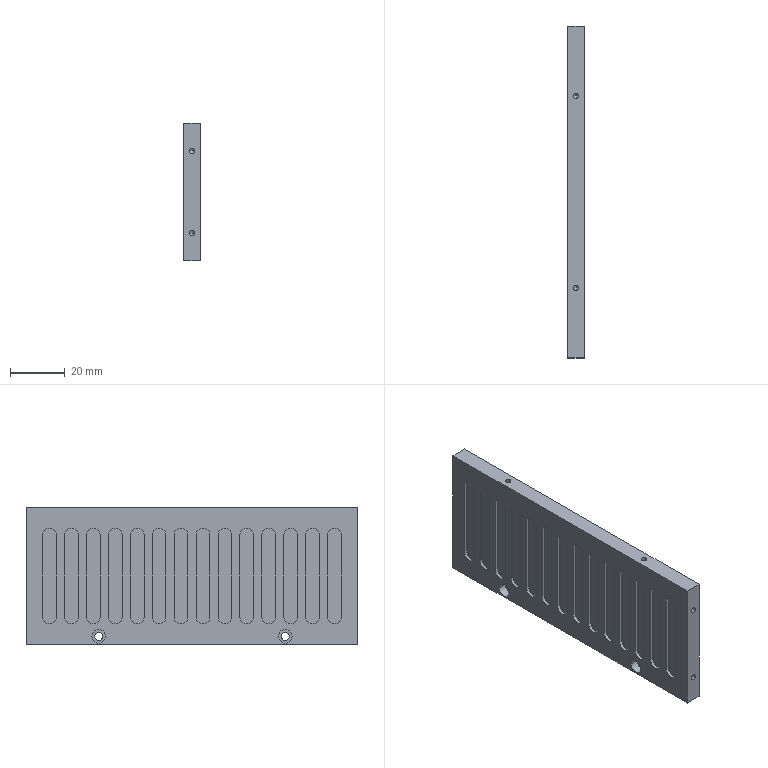CAM job | Mastercam | mm | 6 operations | part box 6 x 121 x 50
1. Helix Bore | 3 - 3 平铣刀
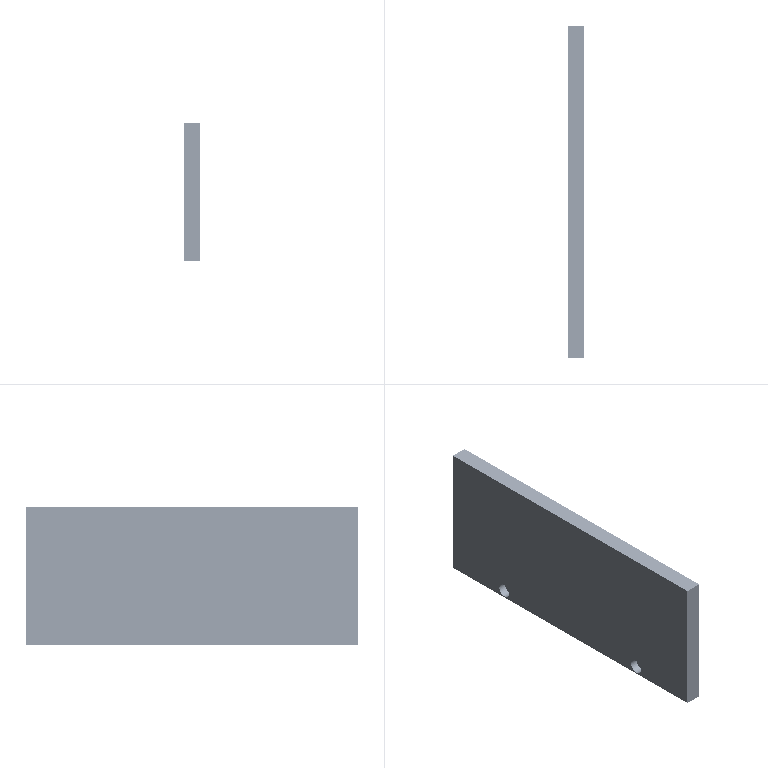2. Contour (Ramp) | 3 - 3 平铣刀
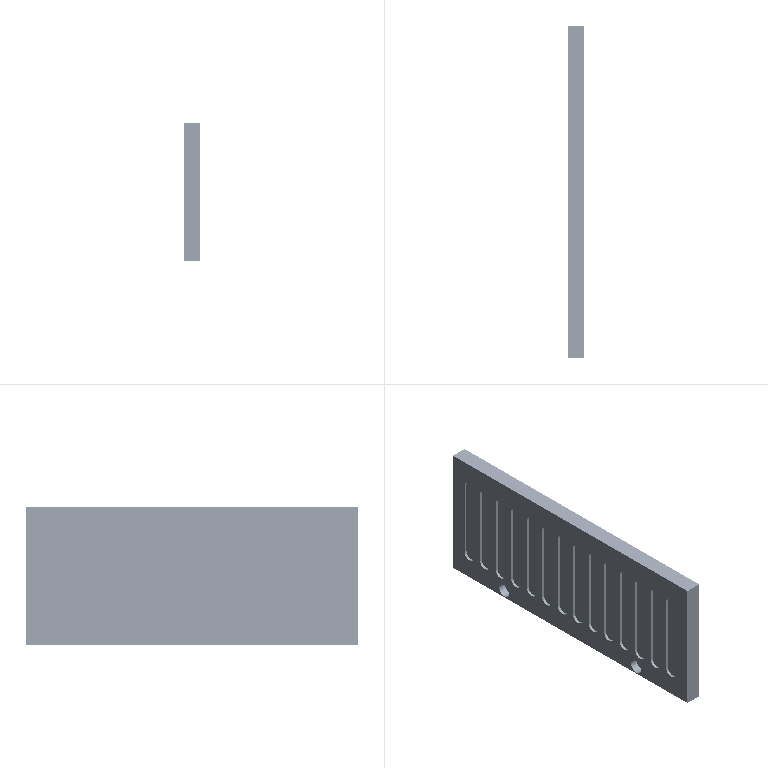3. Contour (2D) | 3 - 3 平铣刀
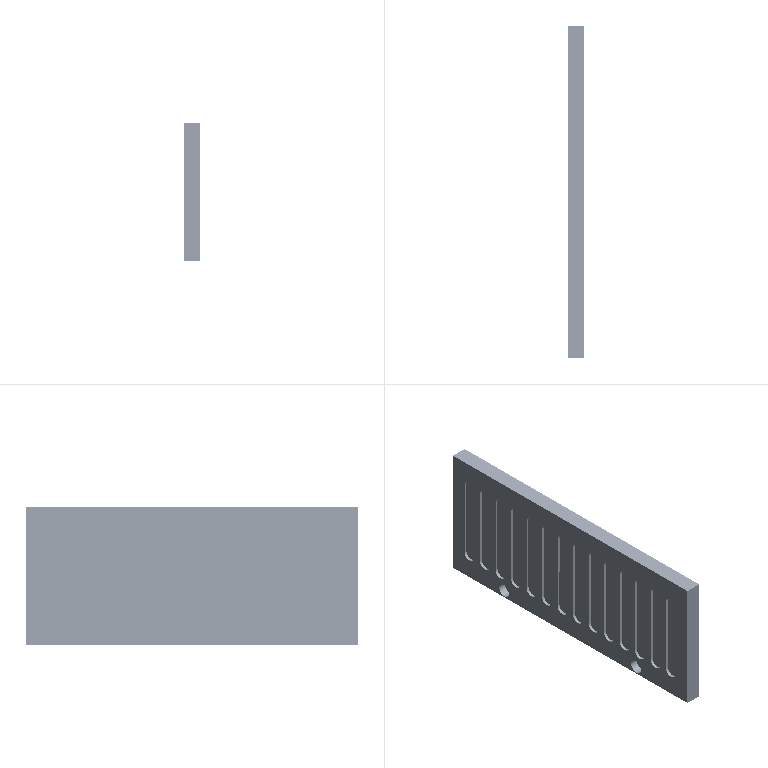4. Contour (2D chamfer) | 5 - 4 倒角刀
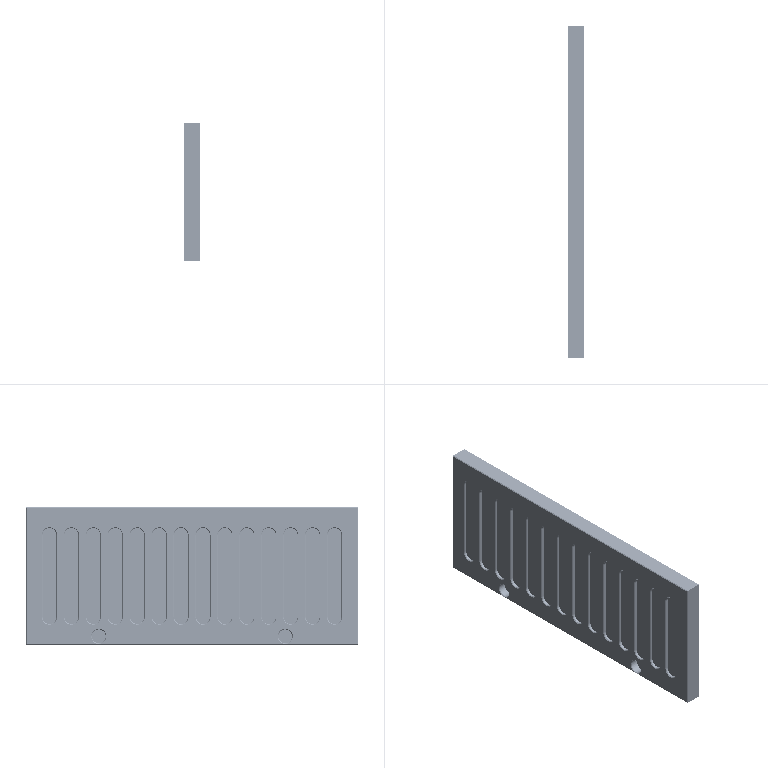5. Drill/Counterbore | 5 - 4 倒角刀
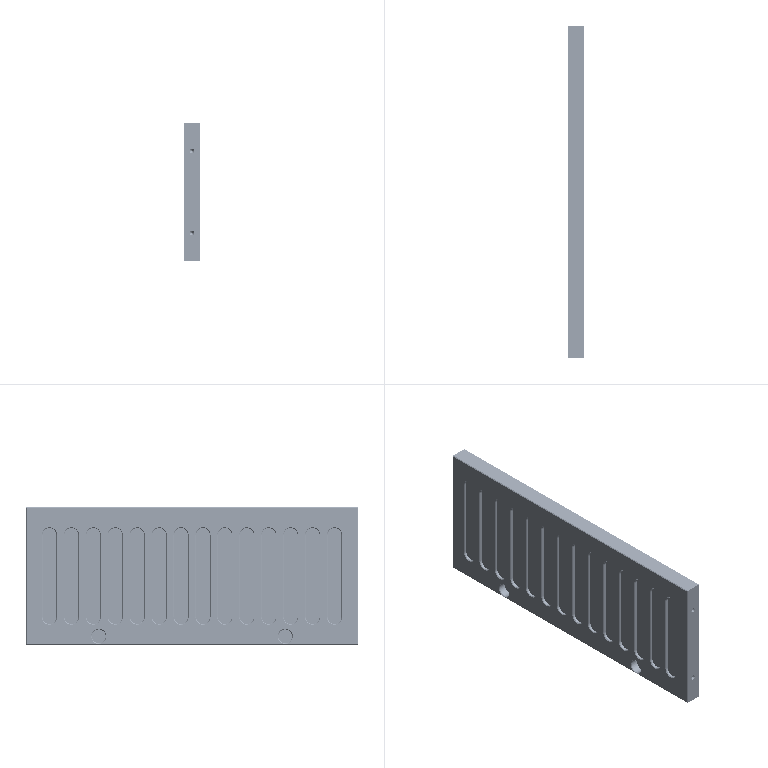6. Drill/Counterbore | 5 - 4 倒角刀